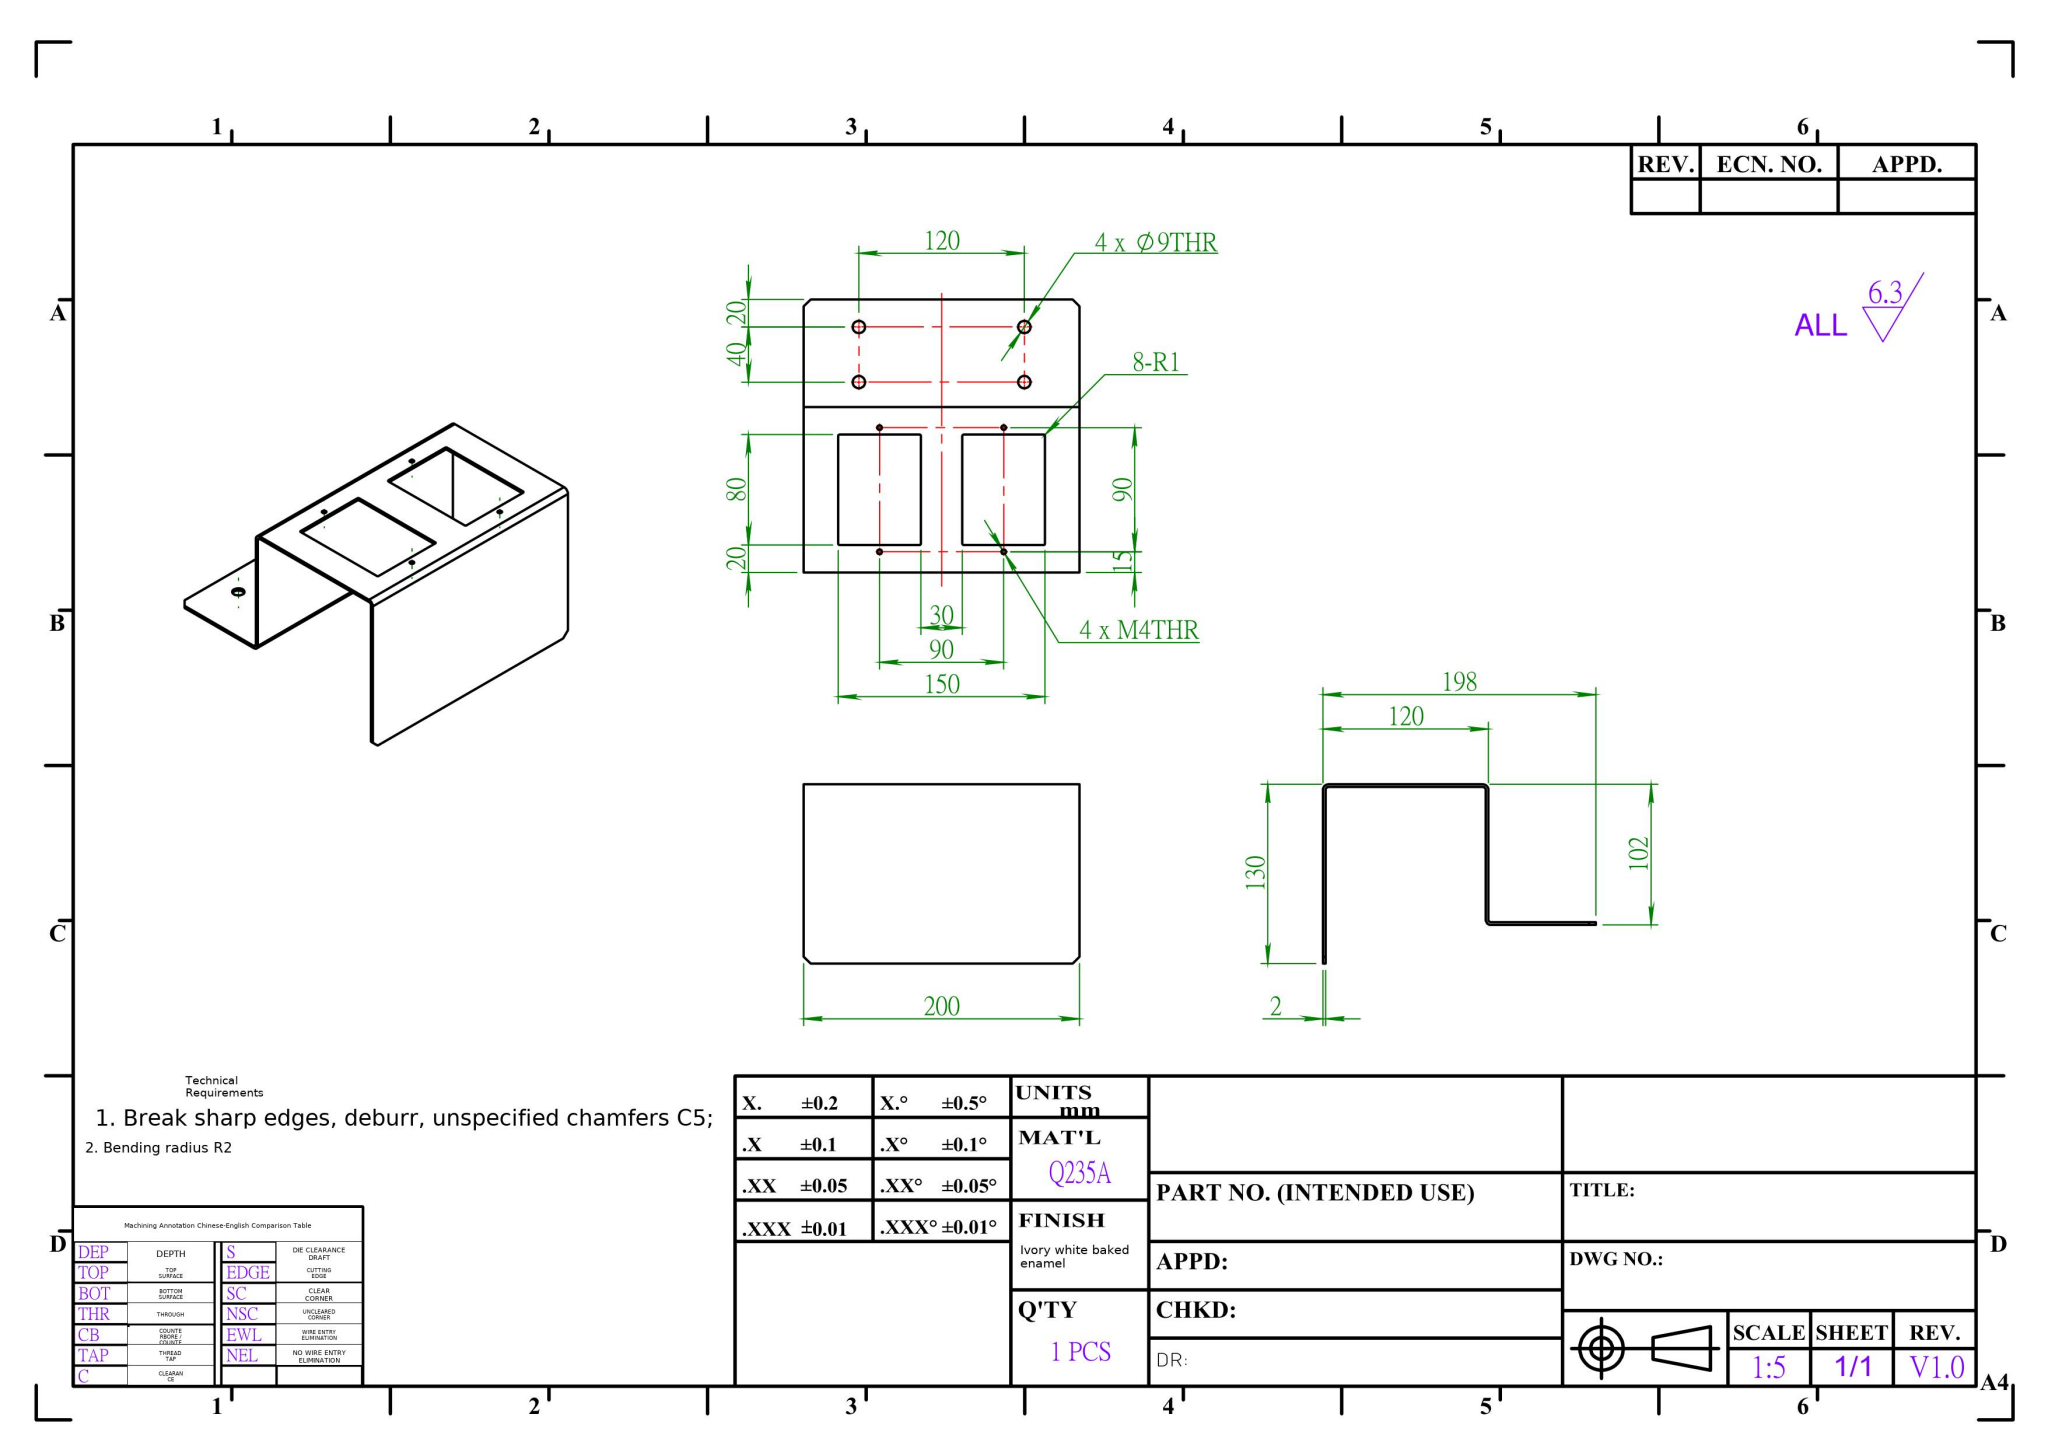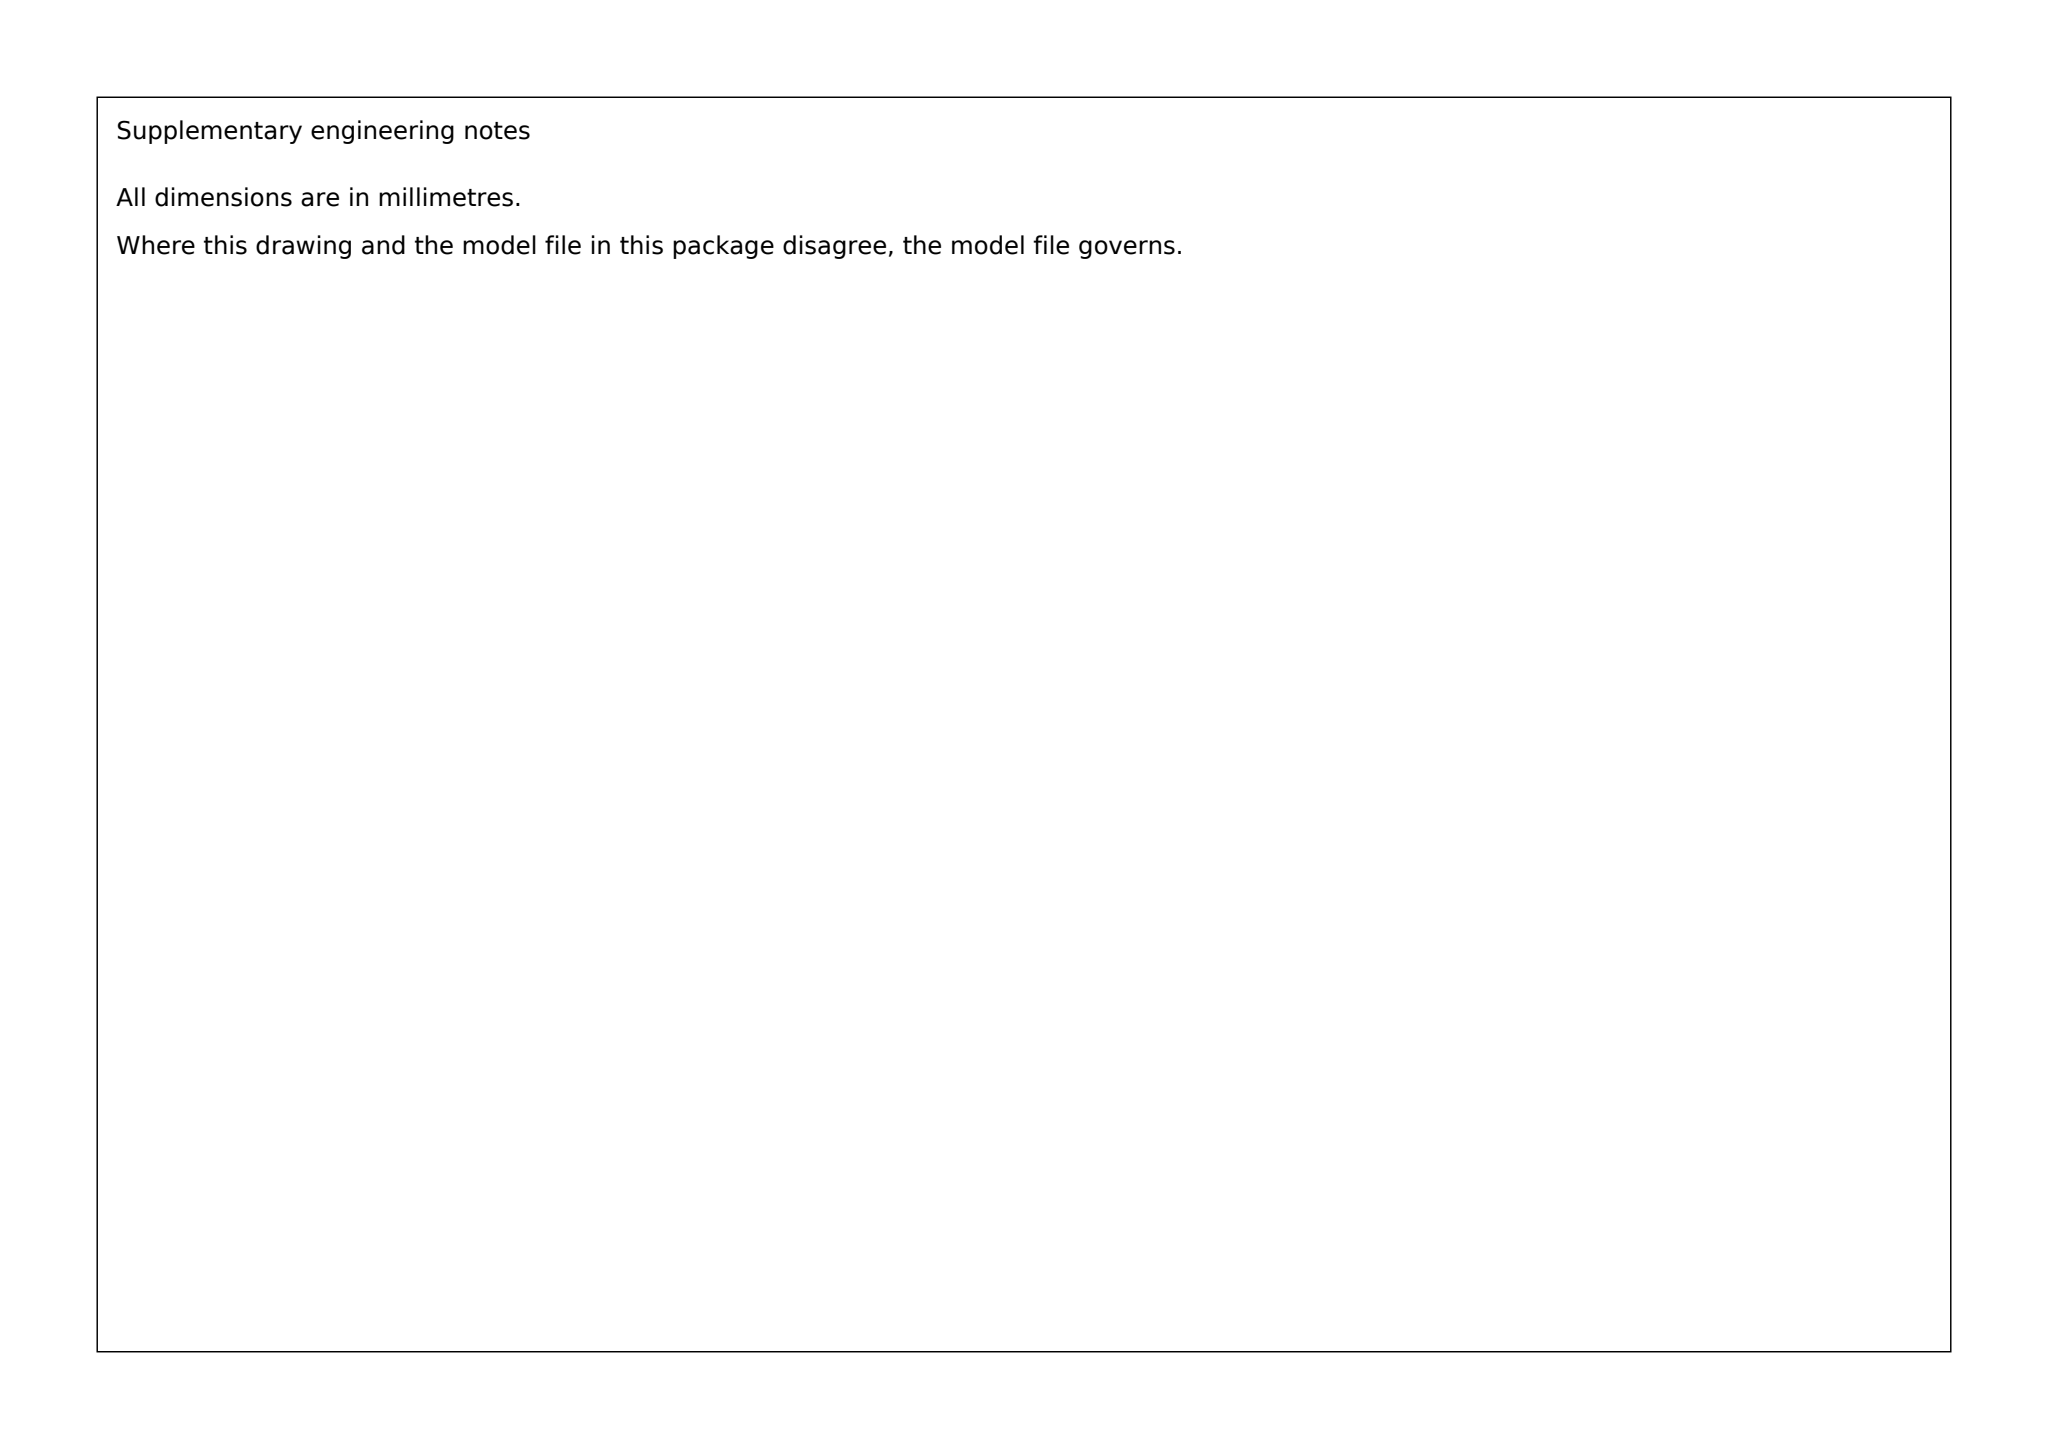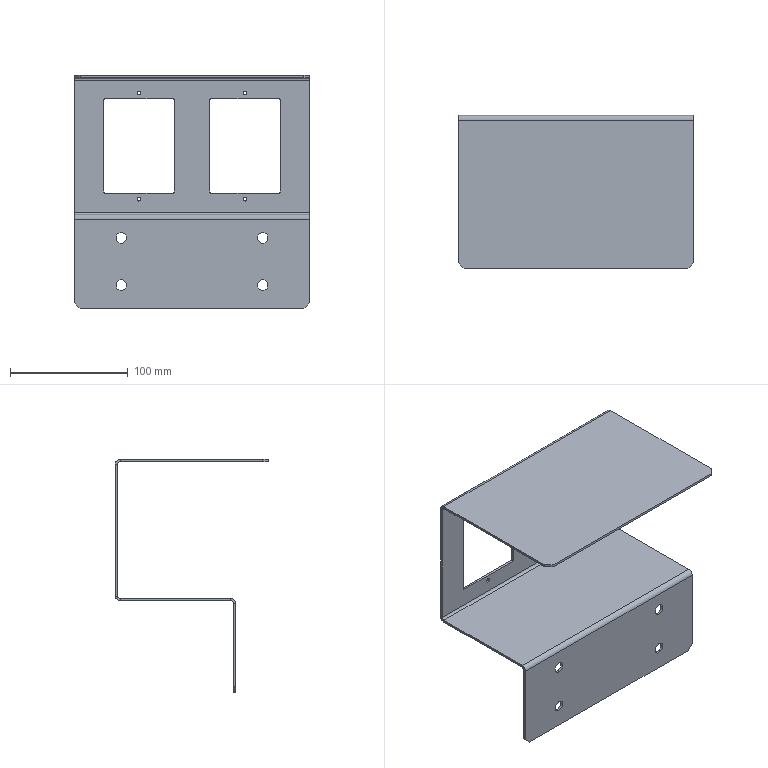Part | SolidWorks | mm | material Q235A | 1 solid | 66 faces | box 200 x 130 x 198 mm | volume 148981 mm3 | plane 36 | cylinder 30 | commonest cylinder face diameters 9 x8 3.3 x8 2 x8 4 x3 8 x3